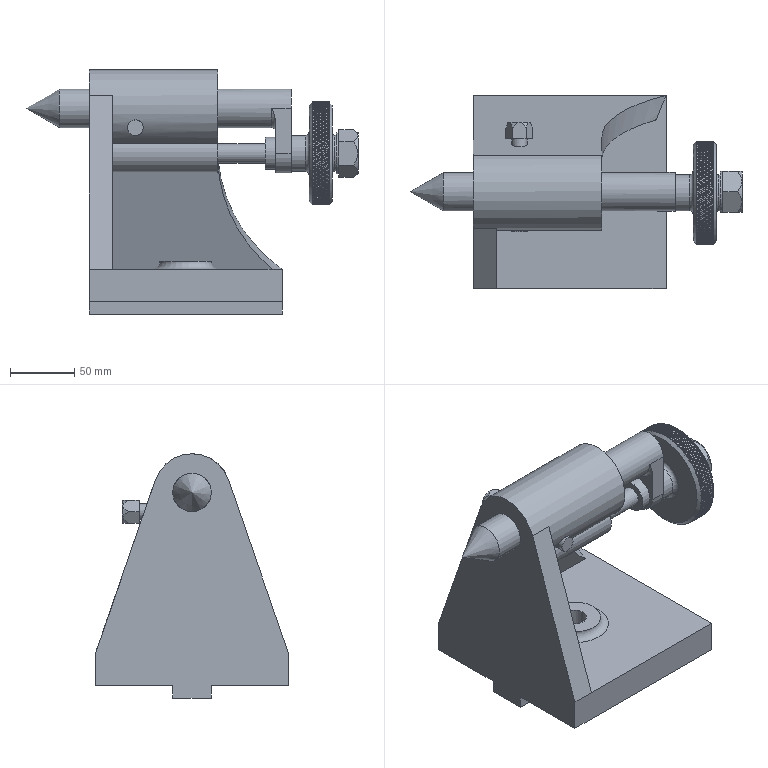Assembly | NX | mm | 8 component files | 8 solids | 2579 faces | box 257.98 x 150 x 190 mm | volume 1550855 mm3 | plane 1801 | cylinder 678 | spline 79 | other 12 | cone 5 | torus 4 | commonest cylinder face diameters 80 x504 15 x61 12 x59 12.1 x24 10.25 x13 30 x6 28 x2 25 x1
Bill of materials:
unnamed part 1 | 1 |  | Hexagonal nut-like body with a central threaded through-bore and chamfered/rounded corners on the hex faces.
unnamed part 2 | 1 |  | Knurled disc/knob with short cylindrical hubs projecting from both faces and a central bore with a single keyway notch.
unnamed part 3 | 1 |  | Plain rectangular bar with square cross-section, like a key or square stock.
unnamed part 4 | 1 |  | Cylindrical shaft with a raised integral collar near mid-length, chamfered ends, and a longitudinal keyway slot on one side of the collar.
unnamed part 5 | 1 |  | Angle bracket/pillow-type mount: rectangular base plate with a raised bossed hole, an upright tapered web topped by a rounded cylindrical boss with a large through-hole and a smaller hole below, a curved gusset on one side, and a small tab projecting below the base.
unnamed part 6 | 1 |  | Thin flat annular ring (plain washer-like disc) with a central round hole.
unnamed part 7 | 1 |  | Hex-head screw/bolt with chamfered head, short plain shank under the head, threaded shank, and a concave cylindrical scallop cut across the threads part-way along the length.
unnamed part 8 | 1 |  | L-shaped pin: straight cylindrical rod with a conical pointed tip at one end and a 90-degree bent flat tab at the other end with a rounded end and a through-hole.
Mates:
1. touch align | centre_head2 1 face | body_1 1 face
2. touch align | screw_4_1 1 face | body_1 1 face
3. touch align | screw_4_1 1 face | centre_head2 1 face
4. parallel | screw_4_1 1 face | centre_head2 1 face
5. distance | centre_head2 1 face | body_1 1 face
6. distance | screw_4_1 1 face | body_1 1 face
7. touch align | hand_wheel 1 face | screw_4_1 1 face
8. distance | hand_wheel 1 face | screw_4_1 1 face
9. touch align | washer_6 1 face | screw_4_1 1 face
10. distance | washer_6 1 face | screw_4_1 1 face
11. touch align | nut_7 1 face | screw_4_1 1 face
12. distance | nut_7 1 face | screw_4_1 1 face